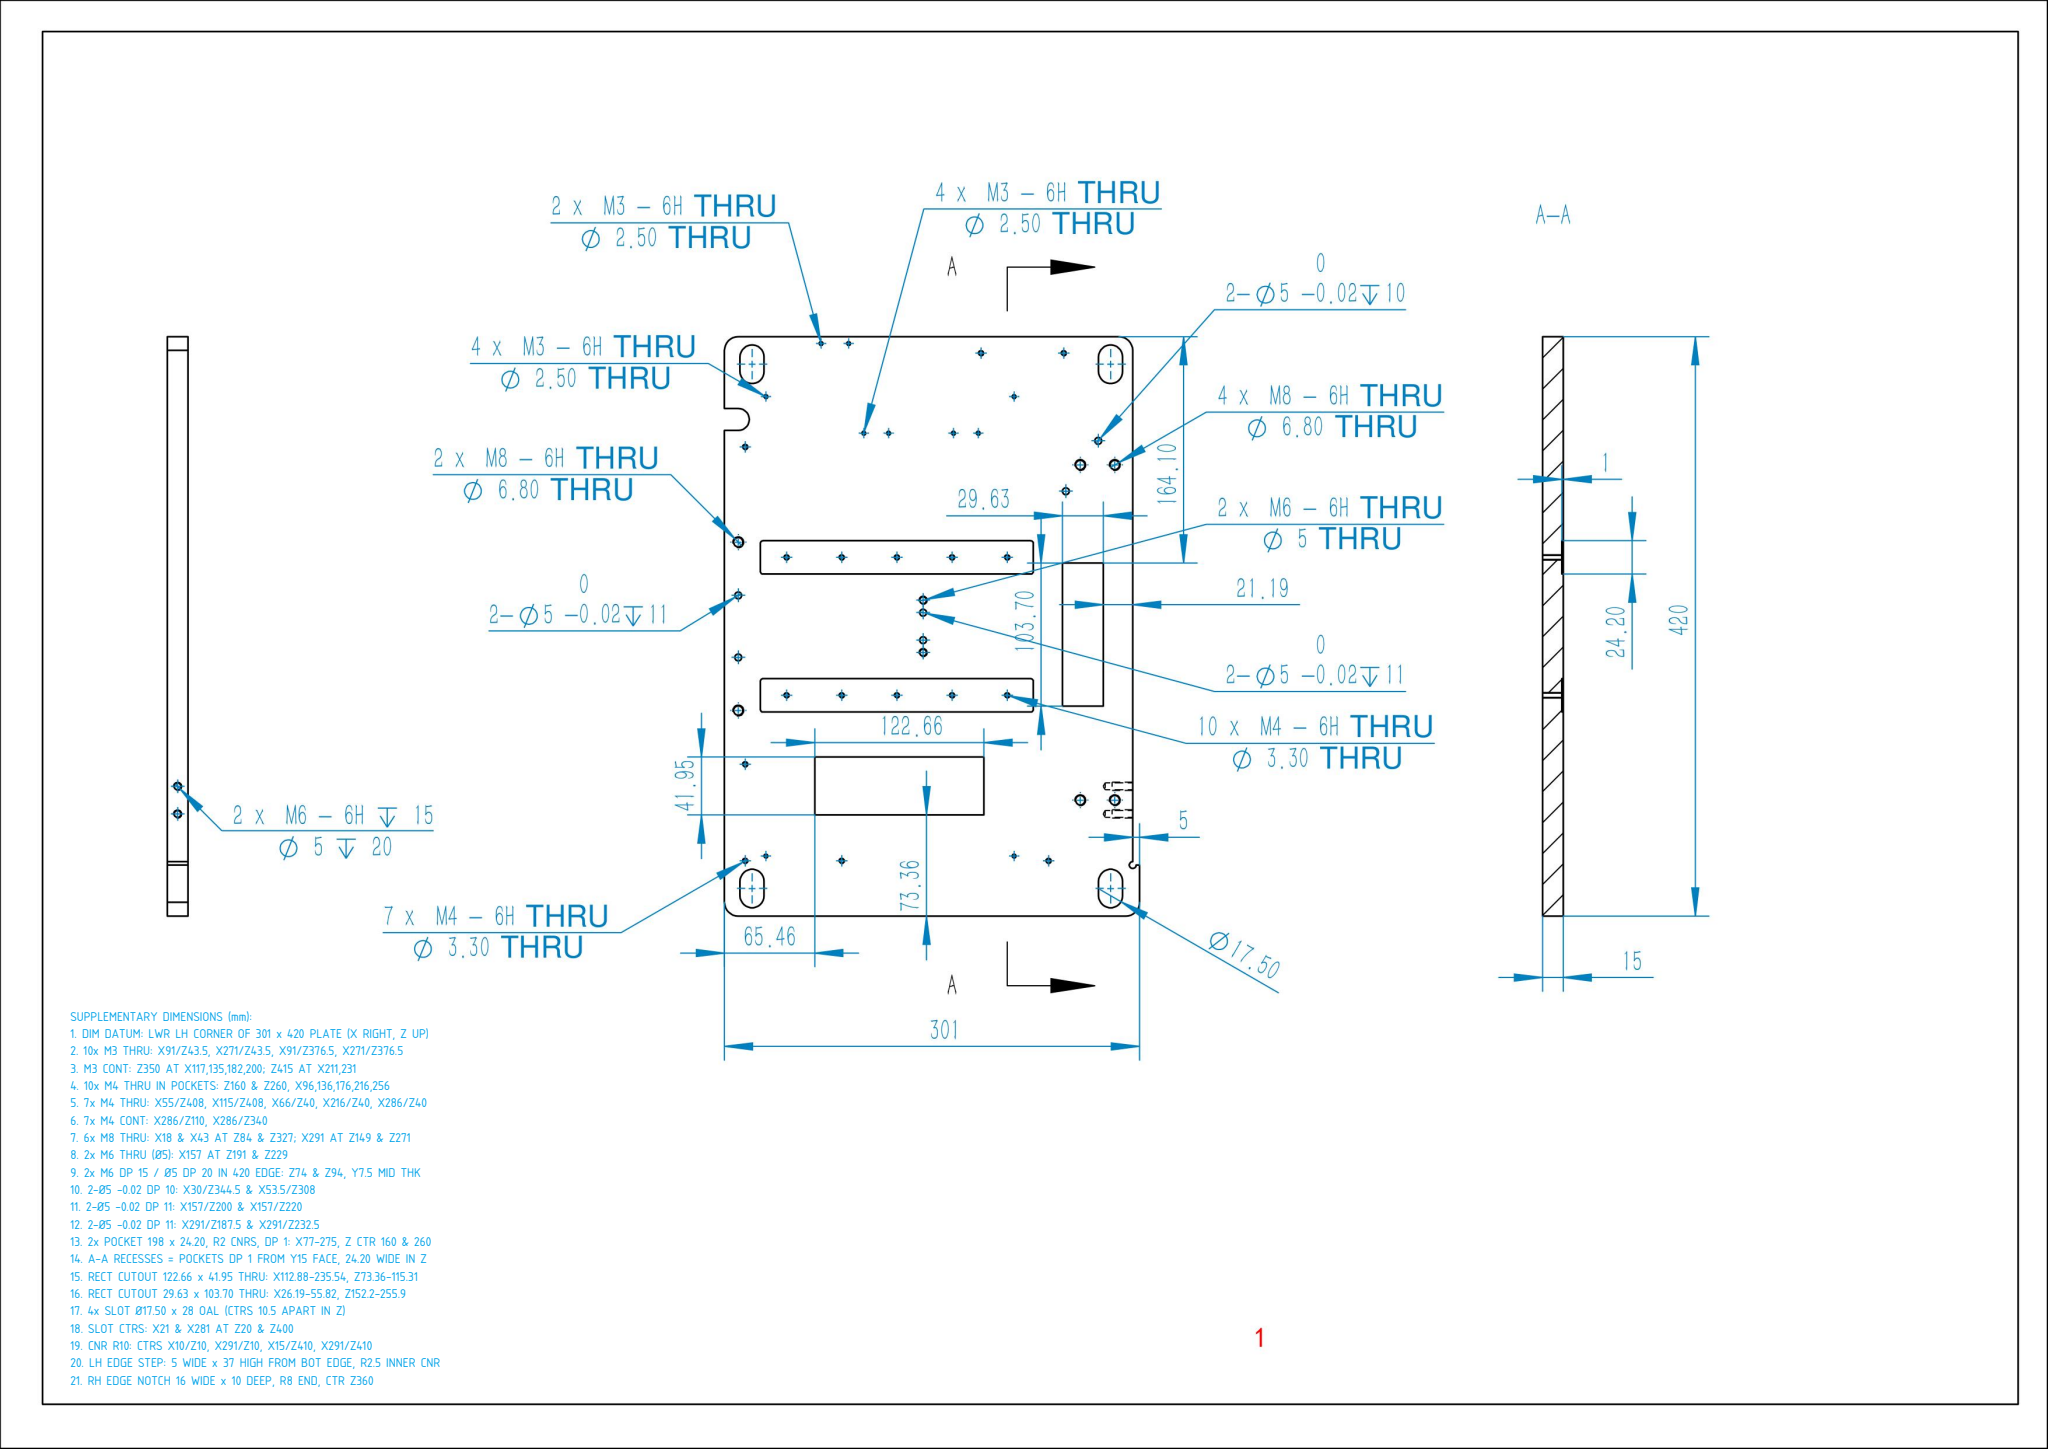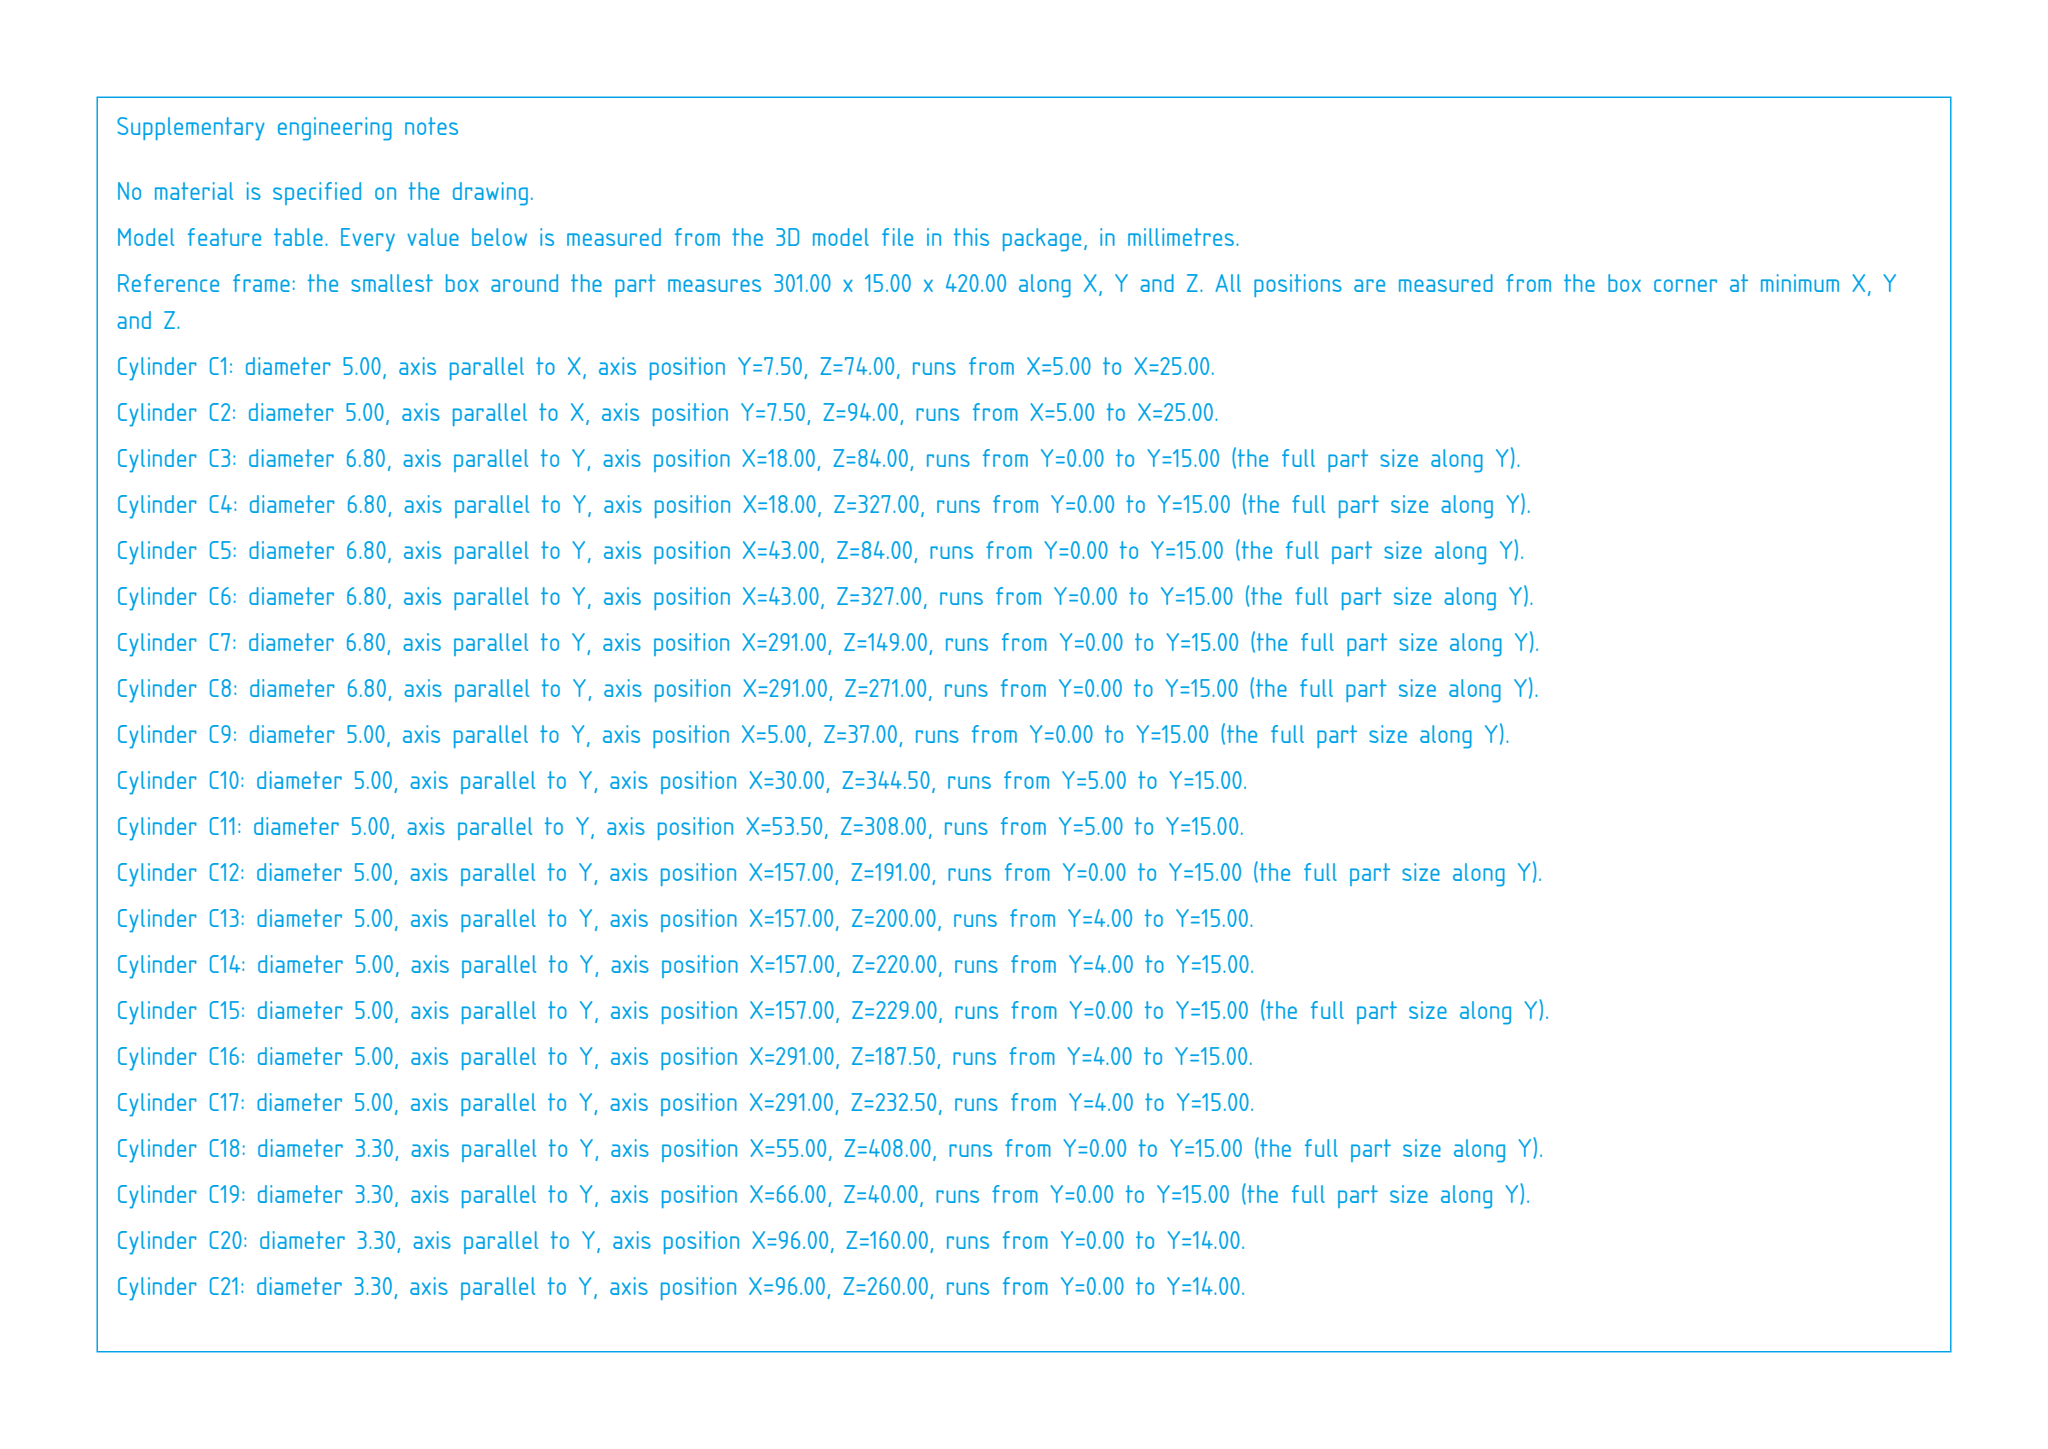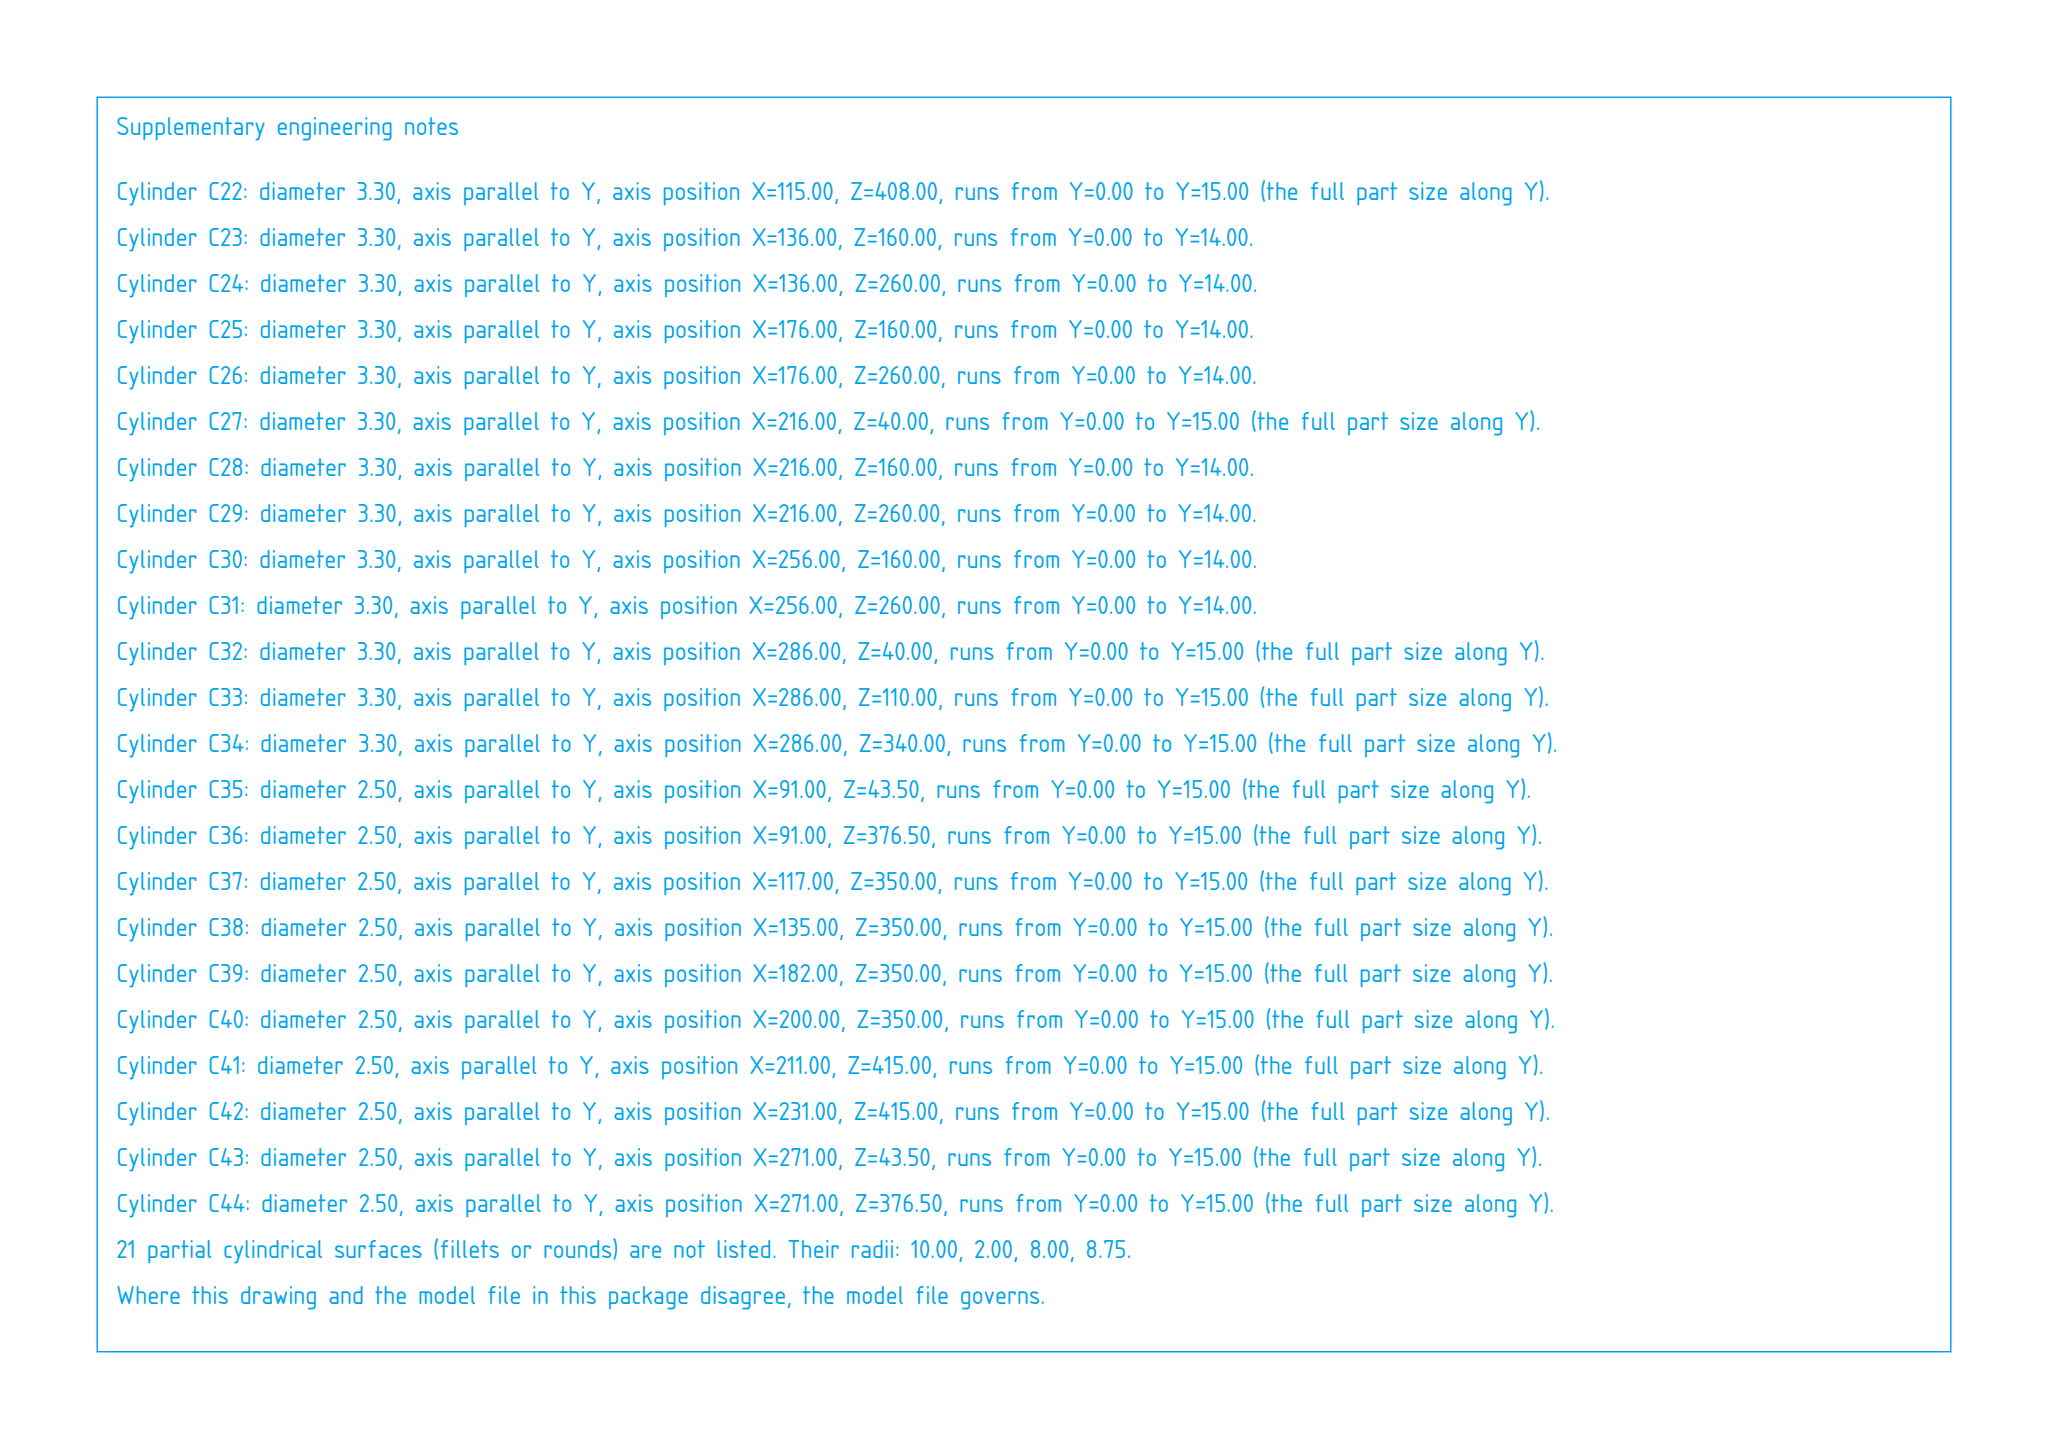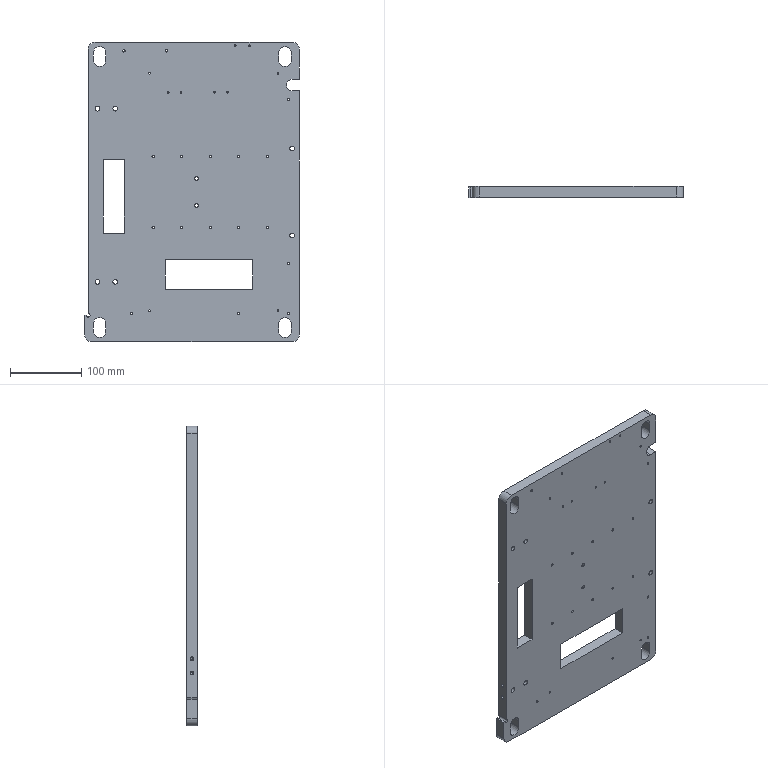Part | SolidWorks | mm | 1 solid | 159 faces | box 301 x 15 x 420 mm | volume 1695097 mm3 | cylinder 112 | plane 43 | cone 4 | commonest cylinder face diameters 3.3 x34 5 x21 2.5 x20 17.5 x12 6.8 x12 4 x8 20 x4 16 x1